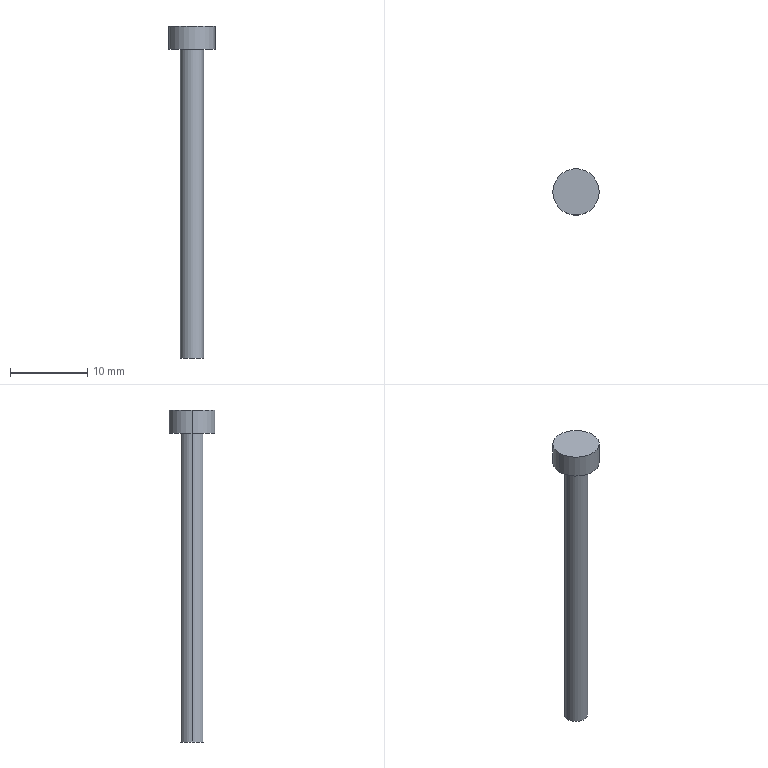Component | SolidWorks | 3mmScrewRod-1 | 1 solid | 7 faces | box 6 x 6 x 43 mm | volume 368 mm3 | cylinder 4 | plane 3 | commonest cylinder face diameters 6 x2 3 x2
build123d program:
from build123d import *

# Parameters (mm, degrees)
SKETCH1_R           = 1.5
BOSS_EXTRUDE1_DEPTH = 20
SKETCH2_R           = 3
BOSS_EXTRUDE2_DEPTH = 3


with BuildPart() as part:
    # Sketch1 → Boss-Extrude1 (new, symmetric)
    with BuildSketch(Plane.XY):
        Circle(SKETCH1_R)
    extrude(amount=BOSS_EXTRUDE1_DEPTH, both=True)

    # Sketch2 → Boss-Extrude2 (add)
    with BuildSketch(Plane.XY.offset(20)):
        Circle(SKETCH2_R)
    extrude(amount=BOSS_EXTRUDE2_DEPTH)


solid = part.part

# Placed as in the assembly
solid = solid.moved(Location((-12.097, -8.483, 39.5), (0, 0, 0)))
STEP:
#1=COLOUR_RGB('',0.7922,0.8196,0.9333);
#2=FILL_AREA_STYLE_COLOUR('',#1);
#3=FILL_AREA_STYLE('',(#2));
#4=SURFACE_STYLE_FILL_AREA(#3);
#5=SURFACE_SIDE_STYLE('',(#4));
#6=SURFACE_STYLE_USAGE(.BOTH.,#5);
#7=PRESENTATION_STYLE_ASSIGNMENT((#6));
#8=CARTESIAN_POINT('',(-0.3581,-0.334,2.461));
#9=VERTEX_POINT('',#8);
#10=CARTESIAN_POINT('',(-0.5944,-0.334,2.461));
#11=VERTEX_POINT('',#10);
#12=CARTESIAN_POINT('',(-0.4763,-0.334,2.461));
#13=DIRECTION('',(0.,0.,1.));
#14=DIRECTION('',(1.,0.,0.));
#15=AXIS2_PLACEMENT_3D('',#12,#13,#14);
#16=CIRCLE('',#15,0.1181);
#17=EDGE_CURVE('',#9,#11,#16,.T.);
#18=ORIENTED_EDGE('',*,*,#17,.F.);
#19=CARTESIAN_POINT('',(-0.3581,-0.334,2.343));
#20=VERTEX_POINT('',#19);
#21=CARTESIAN_POINT('',(-0.3581,-0.334,2.461));
#22=DIRECTION('',(0.,0.,-1.));
#23=VECTOR('',#22,39.37);
#24=LINE('',#21,#23);
#25=EDGE_CURVE('',#9,#20,#24,.T.);
#26=ORIENTED_EDGE('',*,*,#25,.T.);
#27=CARTESIAN_POINT('',(-0.5944,-0.334,2.343));
#28=VERTEX_POINT('',#27);
#29=CARTESIAN_POINT('',(-0.4763,-0.334,2.343));
#30=DIRECTION('',(0.,0.,1.));
#31=DIRECTION('',(1.,0.,0.));
#32=AXIS2_PLACEMENT_3D('',#29,#30,#31);
#33=CIRCLE('',#32,0.1181);
#34=EDGE_CURVE('',#20,#28,#33,.T.);
#35=ORIENTED_EDGE('',*,*,#34,.T.);
#36=CARTESIAN_POINT('',(-0.5944,-0.334,2.461));
#37=DIRECTION('',(0.,0.,-1.));
#38=VECTOR('',#37,39.37);
#39=LINE('',#36,#38);
#40=EDGE_CURVE('',#11,#28,#39,.T.);
#41=ORIENTED_EDGE('',*,*,#40,.F.);
#42=EDGE_LOOP('',(#18,#26,#35,#41));
#43=FACE_OUTER_BOUND('',#42,.T.);
#44=CARTESIAN_POINT('',(-0.4763,-0.334,2.461));
#45=DIRECTION('',(0.,0.,-1.));
#46=DIRECTION('',(-1.,0.,0.));
#47=AXIS2_PLACEMENT_3D('',#44,#45,#46);
#48=CYLINDRICAL_SURFACE('',#47,0.1181);
#49=ADVANCED_FACE('',(#43),#48,.T.);
#50=CARTESIAN_POINT('',(-0.4172,-0.334,2.343));
#51=VERTEX_POINT('',#50);
#52=CARTESIAN_POINT('',(-0.5353,-0.334,2.343));
#53=VERTEX_POINT('',#52);
#54=CARTESIAN_POINT('',(-0.4763,-0.334,2.343));
#55=DIRECTION('',(0.,0.,1.));
#56=DIRECTION('',(1.,0.,0.));
#57=AXIS2_PLACEMENT_3D('',#54,#55,#56);
#58=CIRCLE('',#57,0.05906);
#59=EDGE_CURVE('',#51,#53,#58,.T.);
#60=ORIENTED_EDGE('',*,*,#59,.F.);
#61=CARTESIAN_POINT('',(-0.4172,-0.334,0.7677));
#62=VERTEX_POINT('',#61);
#63=CARTESIAN_POINT('',(-0.4172,-0.334,2.343));
#64=DIRECTION('',(0.,0.,-1.));
#65=VECTOR('',#64,39.37);
#66=LINE('',#63,#65);
#67=EDGE_CURVE('',#51,#62,#66,.T.);
#68=ORIENTED_EDGE('',*,*,#67,.T.);
#69=CARTESIAN_POINT('',(-0.5353,-0.334,0.7677));
#70=VERTEX_POINT('',#69);
#71=CARTESIAN_POINT('',(-0.4763,-0.334,0.7677));
#72=DIRECTION('',(0.,0.,1.));
#73=DIRECTION('',(1.,0.,0.));
#74=AXIS2_PLACEMENT_3D('',#71,#72,#73);
#75=CIRCLE('',#74,0.05906);
#76=EDGE_CURVE('',#62,#70,#75,.T.);
#77=ORIENTED_EDGE('',*,*,#76,.T.);
#78=CARTESIAN_POINT('',(-0.5353,-0.334,2.343));
#79=DIRECTION('',(0.,0.,-1.));
#80=VECTOR('',#79,39.37);
#81=LINE('',#78,#80);
#82=EDGE_CURVE('',#53,#70,#81,.T.);
#83=ORIENTED_EDGE('',*,*,#82,.F.);
#84=EDGE_LOOP('',(#60,#68,#77,#83));
#85=FACE_OUTER_BOUND('',#84,.T.);
#86=CARTESIAN_POINT('',(-0.4763,-0.334,2.343));
#87=DIRECTION('',(0.,0.,-1.));
#88=DIRECTION('',(-1.,0.,0.));
#89=AXIS2_PLACEMENT_3D('',#86,#87,#88);
#90=CYLINDRICAL_SURFACE('',#89,0.05906);
#91=ADVANCED_FACE('',(#85),#90,.T.);
#92=ORIENTED_EDGE('',*,*,#67,.F.);
#93=CARTESIAN_POINT('',(-0.4763,-0.334,2.343));
#94=DIRECTION('',(0.,0.,1.));
#95=DIRECTION('',(1.,0.,0.));
#96=AXIS2_PLACEMENT_3D('',#93,#94,#95);
#97=CIRCLE('',#96,0.05906);
#98=EDGE_CURVE('',#53,#51,#97,.T.);
#99=ORIENTED_EDGE('',*,*,#98,.F.);
#100=ORIENTED_EDGE('',*,*,#82,.T.);
#101=CARTESIAN_POINT('',(-0.4763,-0.334,0.7677));
#102=DIRECTION('',(0.,0.,1.));
#103=DIRECTION('',(1.,0.,0.));
#104=AXIS2_PLACEMENT_3D('',#101,#102,#103);
#105=CIRCLE('',#104,0.05906);
#106=EDGE_CURVE('',#70,#62,#105,.T.);
#107=ORIENTED_EDGE('',*,*,#106,.T.);
#108=EDGE_LOOP('',(#92,#99,#100,#107));
#109=FACE_OUTER_BOUND('',#108,.T.);
#110=CARTESIAN_POINT('',(-0.4763,-0.334,2.343));
#111=DIRECTION('',(0.,0.,-1.));
#112=DIRECTION('',(-1.,0.,0.));
#113=AXIS2_PLACEMENT_3D('',#110,#111,#112);
#114=CYLINDRICAL_SURFACE('',#113,0.05906);
#115=ADVANCED_FACE('',(#109),#114,.T.);
#116=ORIENTED_EDGE('',*,*,#106,.F.);
#117=ORIENTED_EDGE('',*,*,#76,.F.);
#118=EDGE_LOOP('',(#116,#117));
#119=FACE_OUTER_BOUND('',#118,.T.);
#120=CARTESIAN_POINT('',(-0.4763,-0.334,0.7677));
#121=DIRECTION('',(0.,0.,1.));
#122=DIRECTION('',(1.,0.,0.));
#123=AXIS2_PLACEMENT_3D('',#120,#121,#122);
#124=PLANE('',#123);
#125=ADVANCED_FACE('',(#119),#124,.F.);
#126=CARTESIAN_POINT('',(-0.4763,-0.334,2.343));
#127=DIRECTION('',(0.,0.,1.));
#128=DIRECTION('',(1.,0.,0.));
#129=AXIS2_PLACEMENT_3D('',#126,#127,#128);
#130=CIRCLE('',#129,0.1181);
#131=EDGE_CURVE('',#28,#20,#130,.T.);
#132=ORIENTED_EDGE('',*,*,#131,.F.);
#133=ORIENTED_EDGE('',*,*,#34,.F.);
#134=EDGE_LOOP('',(#132,#133));
#135=FACE_OUTER_BOUND('',#134,.T.);
#136=ORIENTED_EDGE('',*,*,#98,.T.);
#137=ORIENTED_EDGE('',*,*,#59,.T.);
#138=EDGE_LOOP('',(#136,#137));
#139=FACE_BOUND('',#138,.T.);
#140=CARTESIAN_POINT('',(-0.4763,-0.334,2.343));
#141=DIRECTION('',(0.,0.,1.));
#142=DIRECTION('',(1.,0.,0.));
#143=AXIS2_PLACEMENT_3D('',#140,#141,#142);
#144=PLANE('',#143);
#145=ADVANCED_FACE('',(#135,#139),#144,.F.);
#146=ORIENTED_EDGE('',*,*,#25,.F.);
#147=CARTESIAN_POINT('',(-0.4763,-0.334,2.461));
#148=DIRECTION('',(0.,0.,1.));
#149=DIRECTION('',(1.,0.,0.));
#150=AXIS2_PLACEMENT_3D('',#147,#148,#149);
#151=CIRCLE('',#150,0.1181);
#152=EDGE_CURVE('',#11,#9,#151,.T.);
#153=ORIENTED_EDGE('',*,*,#152,.F.);
#154=ORIENTED_EDGE('',*,*,#40,.T.);
#155=ORIENTED_EDGE('',*,*,#131,.T.);
#156=EDGE_LOOP('',(#146,#153,#154,#155));
#157=FACE_OUTER_BOUND('',#156,.T.);
#158=CARTESIAN_POINT('',(-0.4763,-0.334,2.461));
#159=DIRECTION('',(0.,0.,-1.));
#160=DIRECTION('',(-1.,0.,0.));
#161=AXIS2_PLACEMENT_3D('',#158,#159,#160);
#162=CYLINDRICAL_SURFACE('',#161,0.1181);
#163=ADVANCED_FACE('',(#157),#162,.T.);
#164=ORIENTED_EDGE('',*,*,#152,.T.);
#165=ORIENTED_EDGE('',*,*,#17,.T.);
#166=EDGE_LOOP('',(#164,#165));
#167=FACE_OUTER_BOUND('',#166,.T.);
#168=CARTESIAN_POINT('',(-0.4763,-0.334,2.461));
#169=DIRECTION('',(0.,0.,1.));
#170=DIRECTION('',(1.,0.,0.));
#171=AXIS2_PLACEMENT_3D('',#168,#169,#170);
#172=PLANE('',#171);
#173=ADVANCED_FACE('',(#167),#172,.T.);
#174=CLOSED_SHELL('',(#49,#91,#115,#125,#145,#163,#173));
#175=MANIFOLD_SOLID_BREP('',#174);
#176=STYLED_ITEM('',(#7),#175);
#177=(LENGTH_UNIT()NAMED_UNIT(*)SI_UNIT($,.METRE.));
#178=LENGTH_MEASURE_WITH_UNIT(LENGTH_MEASURE(0.0254),#177);
#179=DIMENSIONAL_EXPONENTS(1.,0.,0.,0.,0.,0.,0.);
#180=(CONVERSION_BASED_UNIT('',#178)LENGTH_UNIT()NAMED_UNIT(#179));
#181=UNCERTAINTY_MEASURE_WITH_UNIT(LENGTH_MEASURE(0.00001),#180,'','');
#182=(NAMED_UNIT(*)PLANE_ANGLE_UNIT()SI_UNIT($,.RADIAN.));
#183=(NAMED_UNIT(*)SI_UNIT($,.STERADIAN.)SOLID_ANGLE_UNIT());
#184=(GEOMETRIC_REPRESENTATION_CONTEXT(3)GLOBAL_UNCERTAINTY_ASSIGNED_CONTEXT((#181))GLOBAL_UNIT_ASSIGNED_CONTEXT((#180,#182,#183))REPRESENTATION_CONTEXT('',''));
#185=MECHANICAL_DESIGN_GEOMETRIC_PRESENTATION_REPRESENTATION('',(#176),#184);
#186=CARTESIAN_POINT('',(0.,0.,0.));
#187=DIRECTION('',(0.,0.,1.));
#188=DIRECTION('',(1.,0.,0.));
#189=AXIS2_PLACEMENT_3D('',#186,#187,#188);
#190=(LENGTH_UNIT()NAMED_UNIT(*)SI_UNIT($,.METRE.));
#191=LENGTH_MEASURE_WITH_UNIT(LENGTH_MEASURE(0.0254),#190);
#192=DIMENSIONAL_EXPONENTS(1.,0.,0.,0.,0.,0.,0.);
#193=(CONVERSION_BASED_UNIT('',#191)LENGTH_UNIT()NAMED_UNIT(#192));
#194=UNCERTAINTY_MEASURE_WITH_UNIT(LENGTH_MEASURE(0.00001),#193,'','');
#195=(NAMED_UNIT(*)PLANE_ANGLE_UNIT()SI_UNIT($,.RADIAN.));
#196=(NAMED_UNIT(*)SI_UNIT($,.STERADIAN.)SOLID_ANGLE_UNIT());
#197=(GEOMETRIC_REPRESENTATION_CONTEXT(3)GLOBAL_UNCERTAINTY_ASSIGNED_CONTEXT((#194))GLOBAL_UNIT_ASSIGNED_CONTEXT((#193,#195,#196))REPRESENTATION_CONTEXT('',''));
#198=ADVANCED_BREP_SHAPE_REPRESENTATION('',(#175,#189),#197);
#199=PRESENTATION_LAYER_ASSIGNMENT('','',(#176));